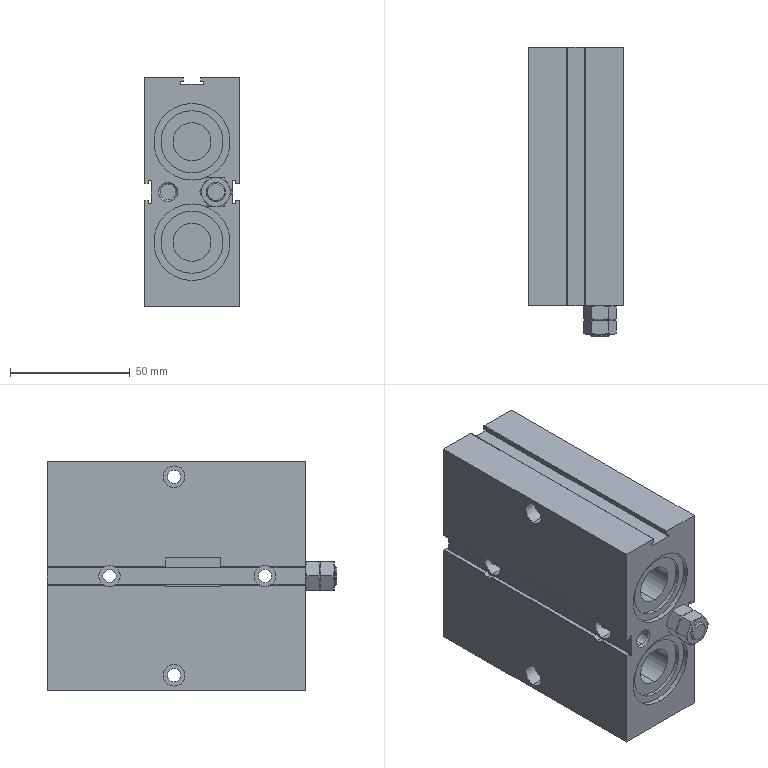Component | SolidWorks | TN32X30S(0)+(CS1-J-1).1-1_TN32-30 - 30_b.1-1 | 1 solid | 235 faces | volume 283820 mm3 | cylinder 112 | plane 91 | cone 32 | commonest cylinder face diameters 0.4 x44 9 x28 32 x12 26 x8 5.5 x8 8.566 x4 16 x4 6.647 x2